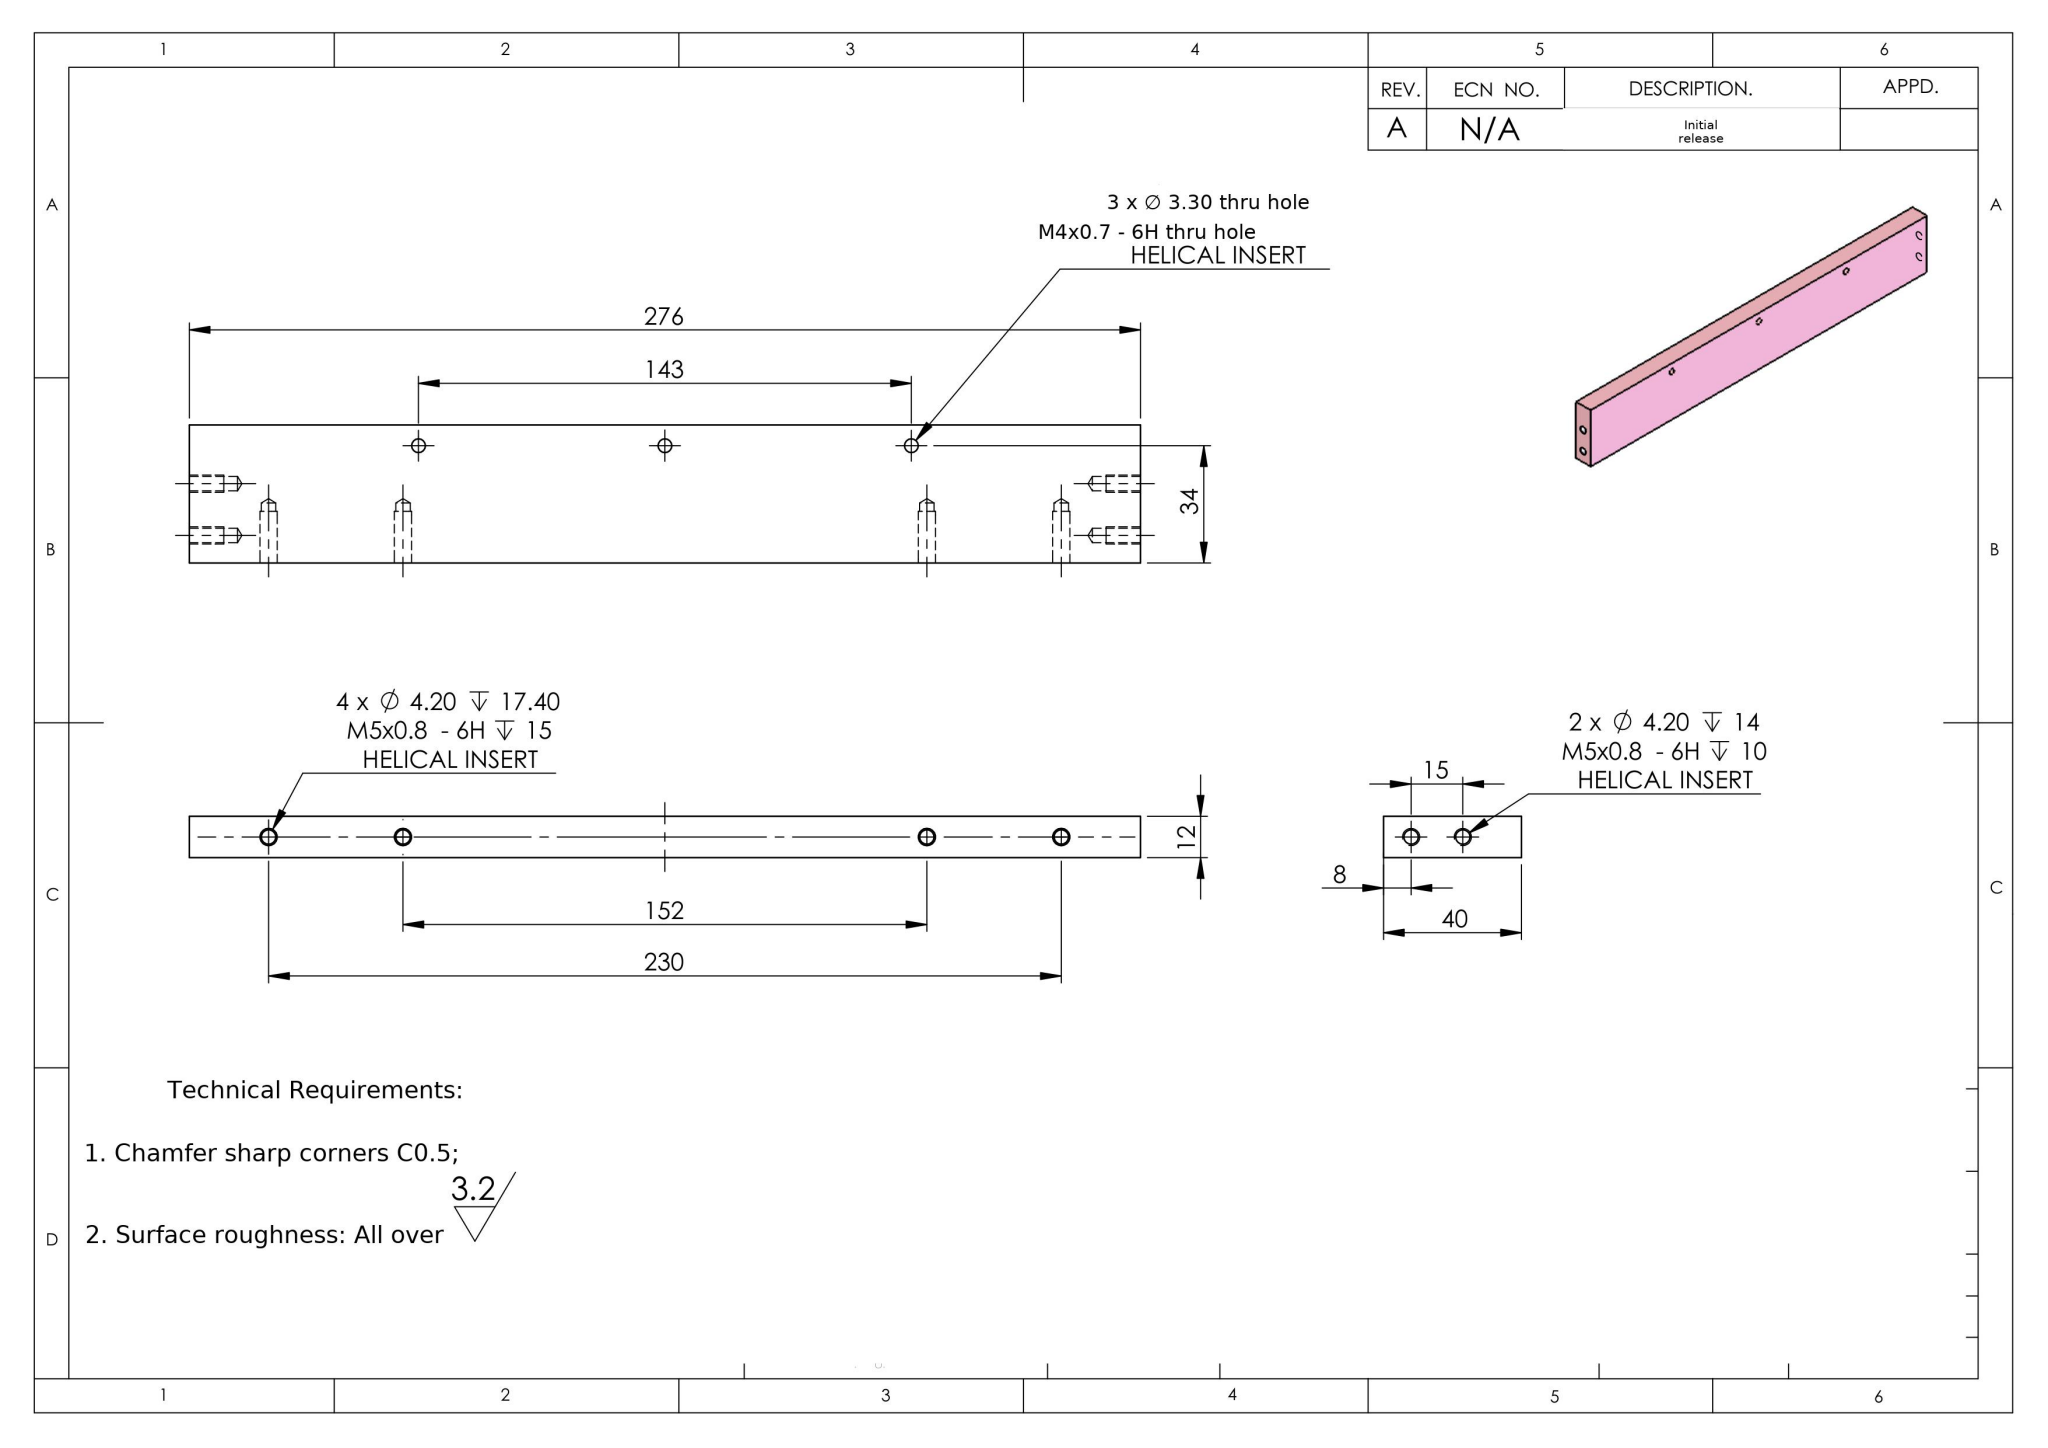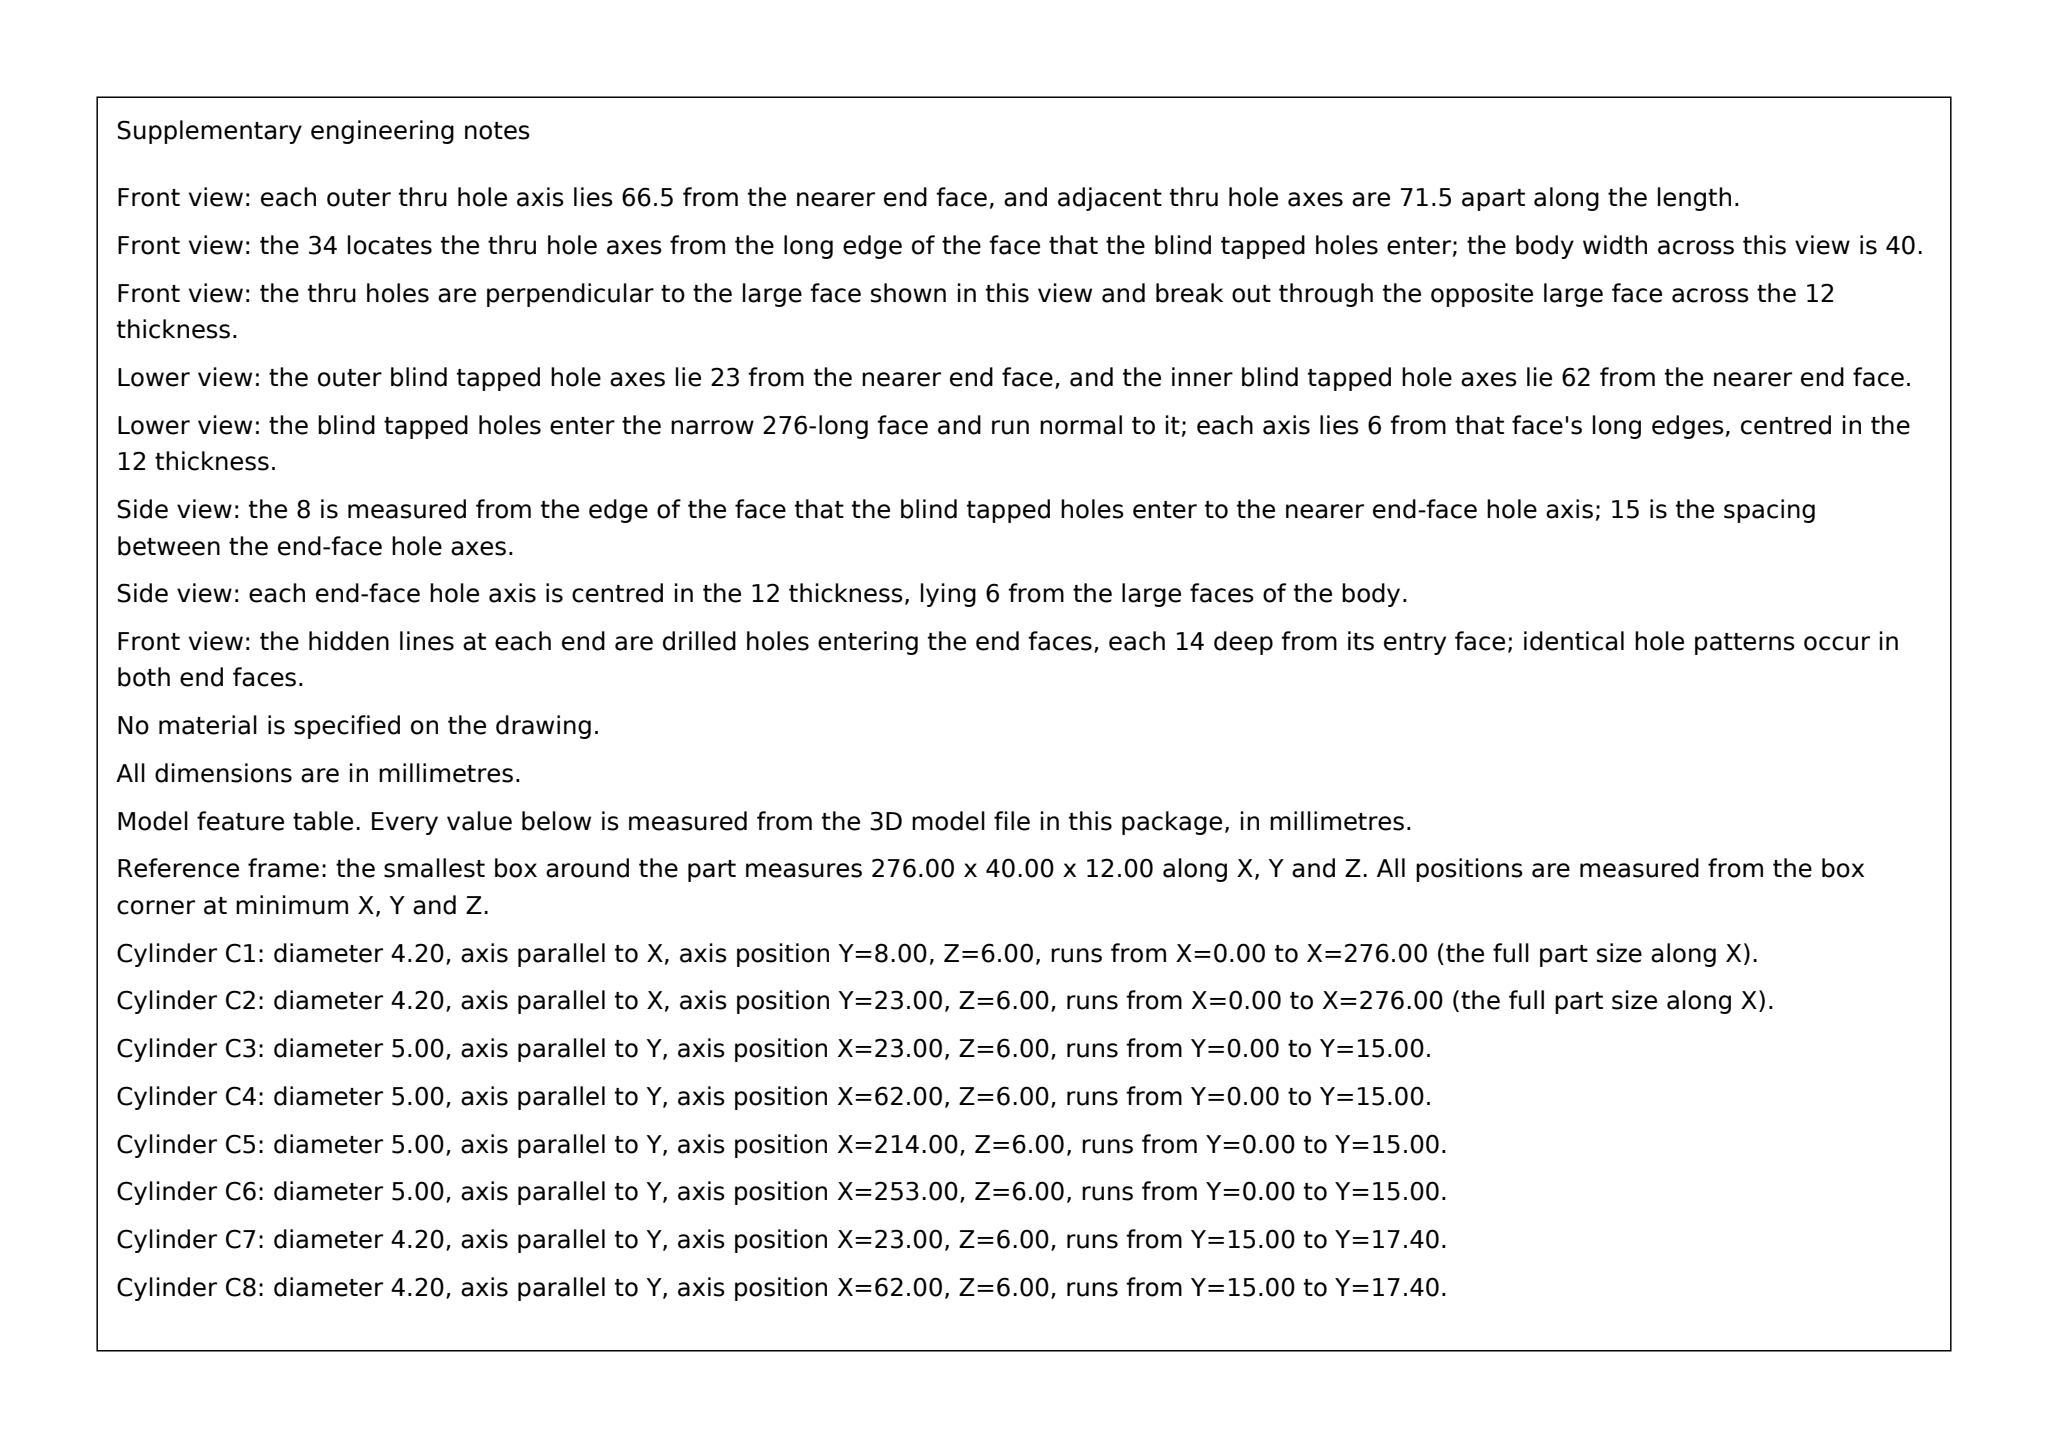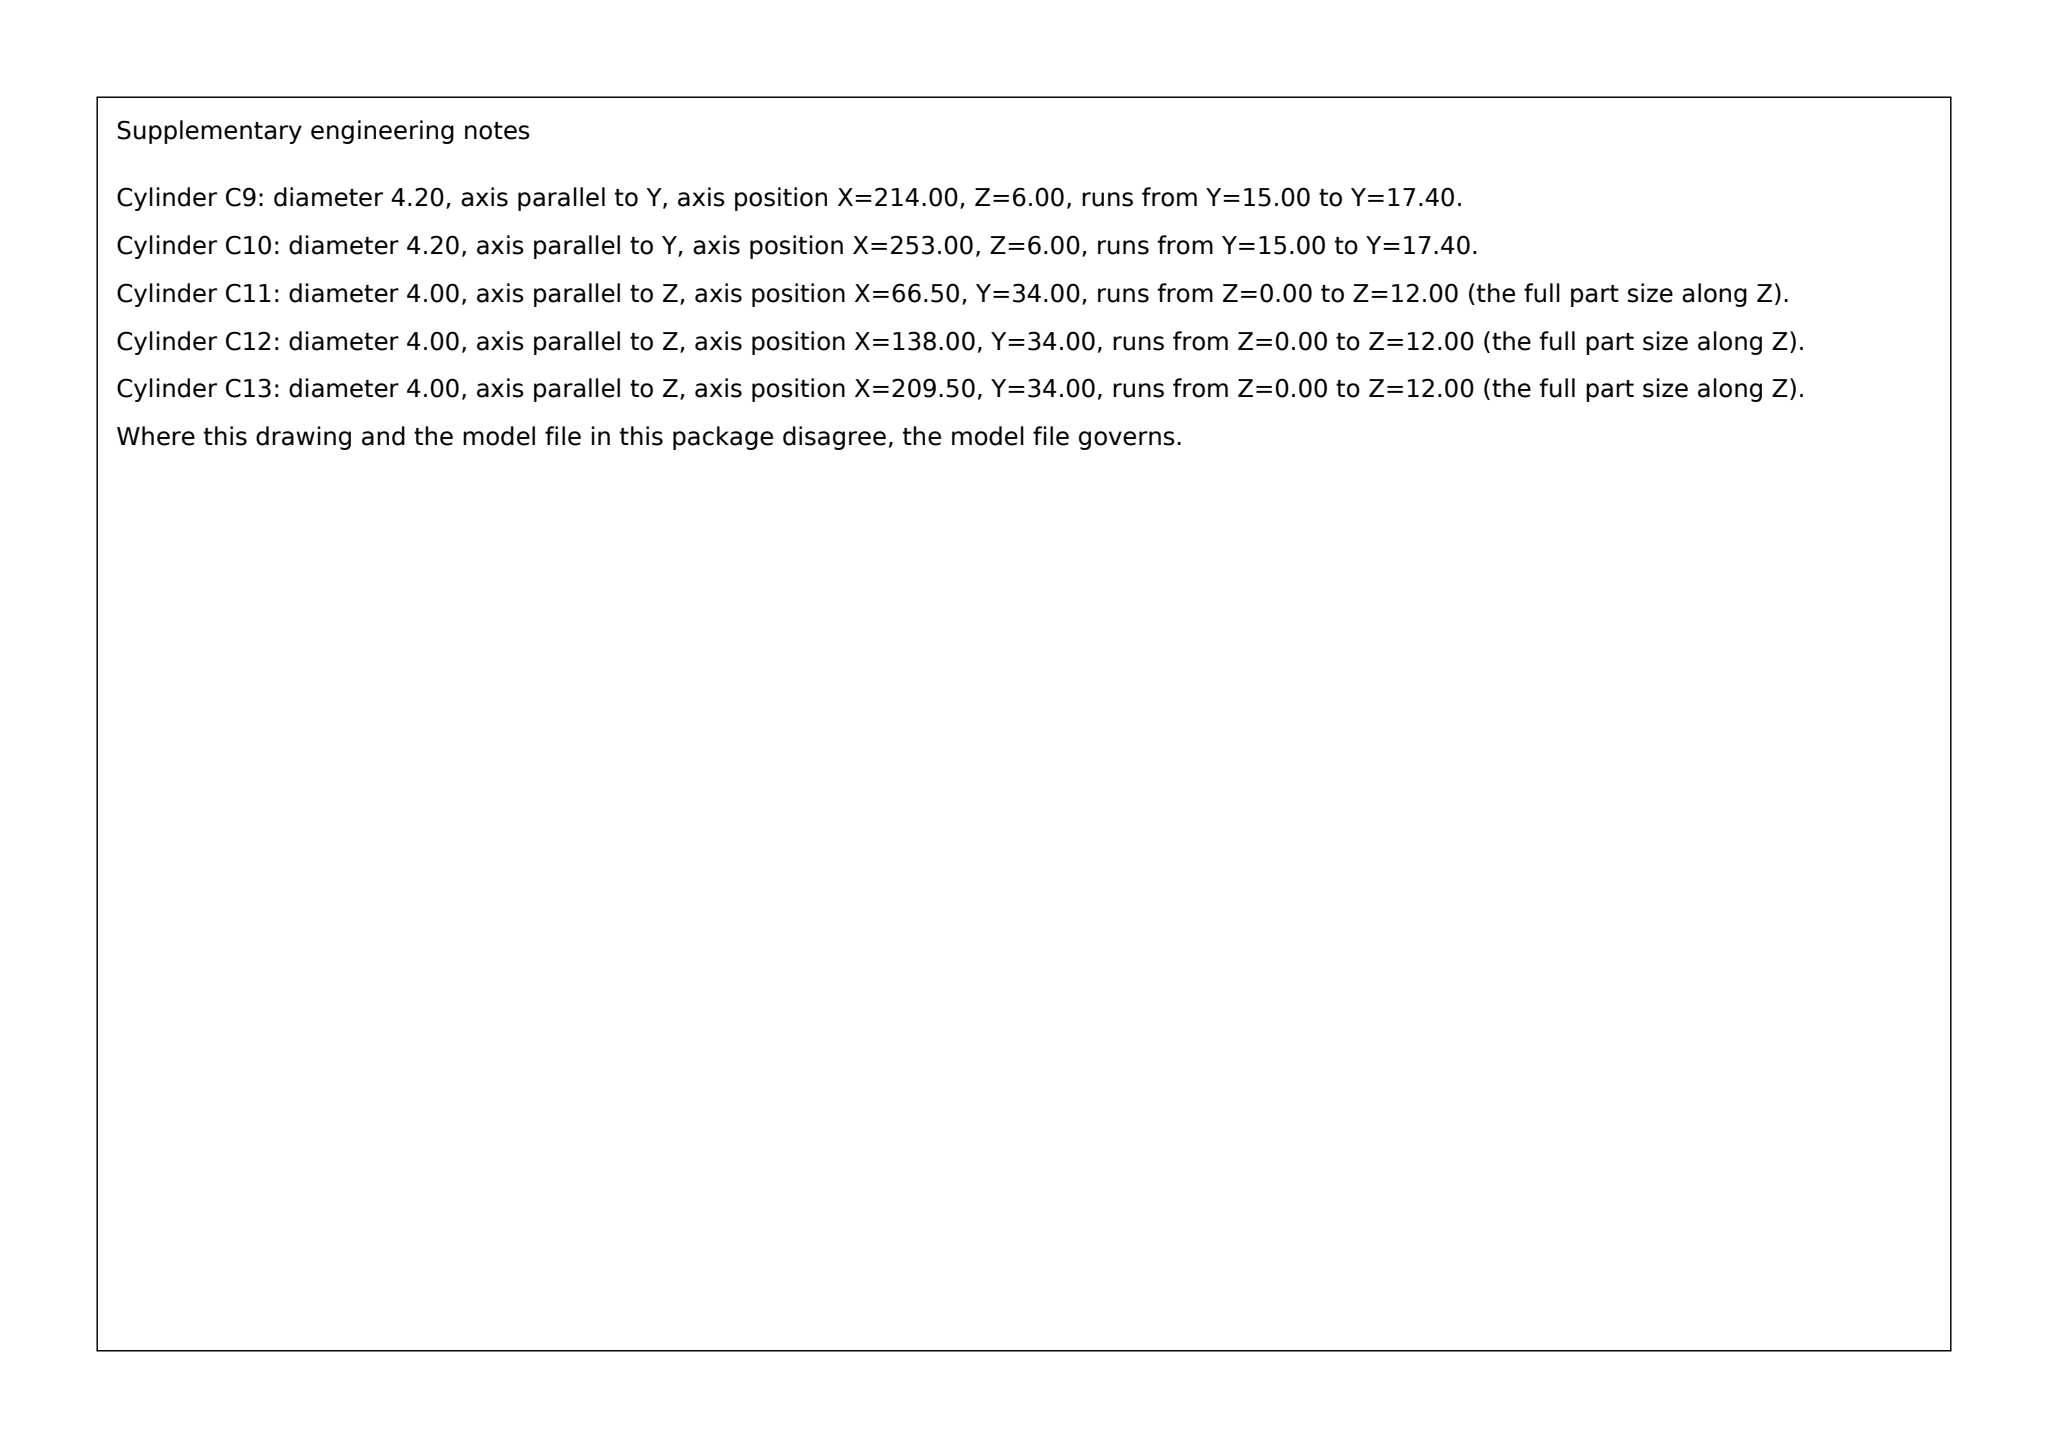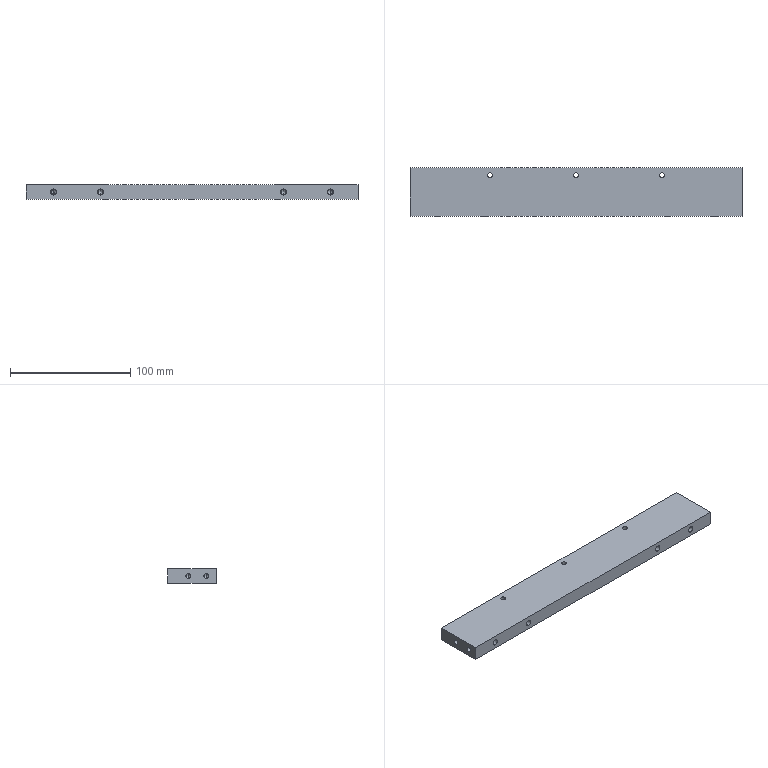Part | SolidWorks | mm | 1 solid | 56 faces | box 276 x 40 x 12 mm | volume 129894 mm3 | cylinder 30 | cone 16 | plane 10 | commonest cylinder face diameters 4.2 x16 5 x8 4 x6
Drawing notes:
3 x M4 THRU: 66.5 FROM LH END FACE, 71.5 EQ SP, SYM ABOUT CL | from the solid: Ø4.0 z-axis holes at x=66.5, 138, 209.5 (y=34), bbox X=276; symmetric about x=138
4 x M5 DP 15 IN SIDE FACE: 23 FROM LH END FACE, SYM ABOUT CL | from the solid: Ø4.2/Ø5.0 y-axis holes at x=23, 62, 214, 253 (z=6); spans 230 & 152, sym about x=138
2 x M5 DP 10 IN END FACE ON 12 THK CL: 6 FROM EA FACE | from the solid: Ø4.2 x-axis holes at z=6.0, thickness planes z=0 and z=12
4 X Ø 4.20 DP 14 / M5X0.8-6H DP 10 HELICAL INSERT, BOTH END FACES | from the solid: Ø4.2 x-axis cyls, L=14, at y=8 & y=23, z=6, count 4 (2 per end face); Ø5 c'bore not present, thread depth per existing note
RH END FACE 2 X M5 SAME AS LH: 8 & 23 FROM BOTTOM EDGE, 15 APART | from the solid: x-axis Ø4.2 holes at y=8.0 and y=23.0 (40 wide face, 15 spacing) at both x=0 and x=276 faces
build123d program:
from build123d import *

# Parameters (mm, degrees)
SKETCH1_W                   = 276
SKETCH1_H                   = 40
EXTRUDE1_DEPTH              = 12
M5_TAPPED_HOLE1_D           = 4.2
M5_TAPPED_HOLE1_DEPTH       = 17.4
M5_TAPPED_HOLE1_CBORE_D     = 5
M5_TAPPED_HOLE1_CBORE_DEPTH = 15
M5_TAPPED_HOLE1_TIP         = 1.262
M5_TAPPED_HOLE2_D           = 4.2
M5_TAPPED_HOLE2_DEPTH       = 14
M5_TAPPED_HOLE2_TIP         = 1.262
M5_TAPPED_HOLE4_D           = 4.2
M5_TAPPED_HOLE4_DEPTH       = 14
M5_TAPPED_HOLE4_TIP         = 1.262
M4_TAPPED_HOLE1_D           = 4


with BuildPart() as part:
    # Sketch1 → Extrude1 (new body)
    with BuildSketch(Plane.XY):
        with Locations((138, 20)):
            Rectangle(SKETCH1_W, SKETCH1_H)
    extrude(amount=EXTRUDE1_DEPTH)

    # M5 Tapped Hole1
    with Locations(Plane.XZ):
        with Locations((62, 6), (214, 6), (23, 6), (253, 6)):
            CounterBoreHole(M5_TAPPED_HOLE1_D / 2, M5_TAPPED_HOLE1_CBORE_D / 2, M5_TAPPED_HOLE1_CBORE_DEPTH, depth=M5_TAPPED_HOLE1_DEPTH)
            with Locations((0, 0, -(M5_TAPPED_HOLE1_DEPTH + M5_TAPPED_HOLE1_TIP / 2))):  # 118° drill point
                Cone(0, M5_TAPPED_HOLE1_D / 2, M5_TAPPED_HOLE1_TIP, mode=Mode.SUBTRACT)

    # M5 Tapped Hole2
    with Locations(Plane.ZY):
        with Locations((6, 8), (6, 23)):
            Hole(M5_TAPPED_HOLE2_D / 2, depth=M5_TAPPED_HOLE2_DEPTH)
            with Locations((0, 0, -(M5_TAPPED_HOLE2_DEPTH + M5_TAPPED_HOLE2_TIP / 2))):  # 118° drill point
                Cone(0, M5_TAPPED_HOLE2_D / 2, M5_TAPPED_HOLE2_TIP, mode=Mode.SUBTRACT)

    # M5 Tapped Hole4
    with Locations(Plane(origin=(276, 0, 0), x_dir=(0, 0, -1), z_dir=(1, 0, 0))):
        with Locations((-6, 8), (-6, 23)):
            Hole(M5_TAPPED_HOLE4_D / 2, depth=M5_TAPPED_HOLE4_DEPTH)
            with Locations((0, 0, -(M5_TAPPED_HOLE4_DEPTH + M5_TAPPED_HOLE4_TIP / 2))):  # 118° drill point
                Cone(0, M5_TAPPED_HOLE4_D / 2, M5_TAPPED_HOLE4_TIP, mode=Mode.SUBTRACT)

    # M4 Tapped Hole1 (through all)
    with Locations(Plane(origin=(209.5, 34, 12), x_dir=(1, 0, 0), z_dir=(0, 0, 1))):
        with Locations((0, 0), (-71.5, 0), (-143, 0)):
            Hole(M4_TAPPED_HOLE1_D / 2)


solid = part.part